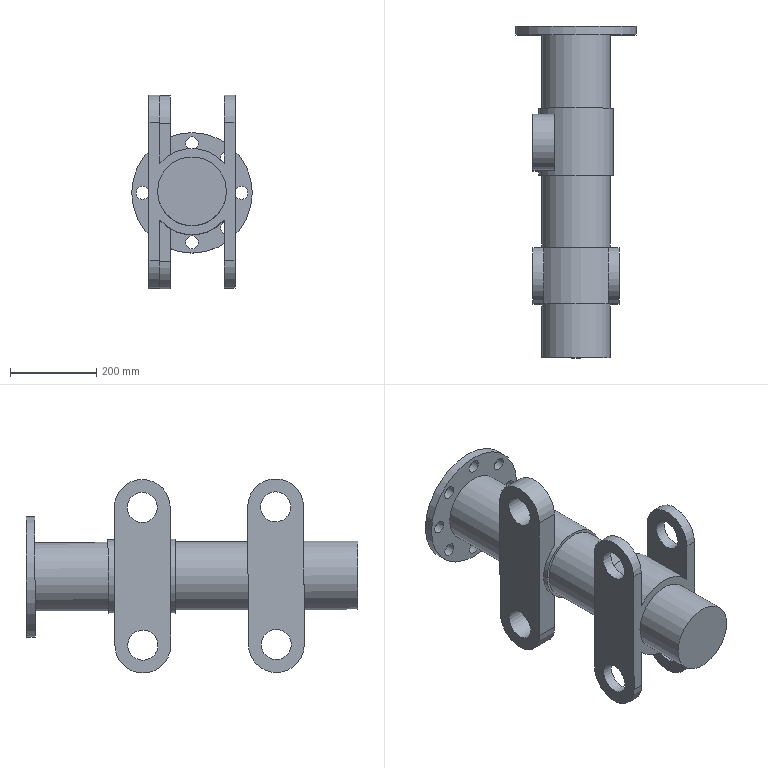Component | NX | COLUMN | 1 solid | 45 faces | volume 21857432 mm3 | cylinder 27 | plane 18 | commonest cylinder face diameters 30 x8 130 x6 70 x6 160 x3 200 x2 173 x1 280 x1